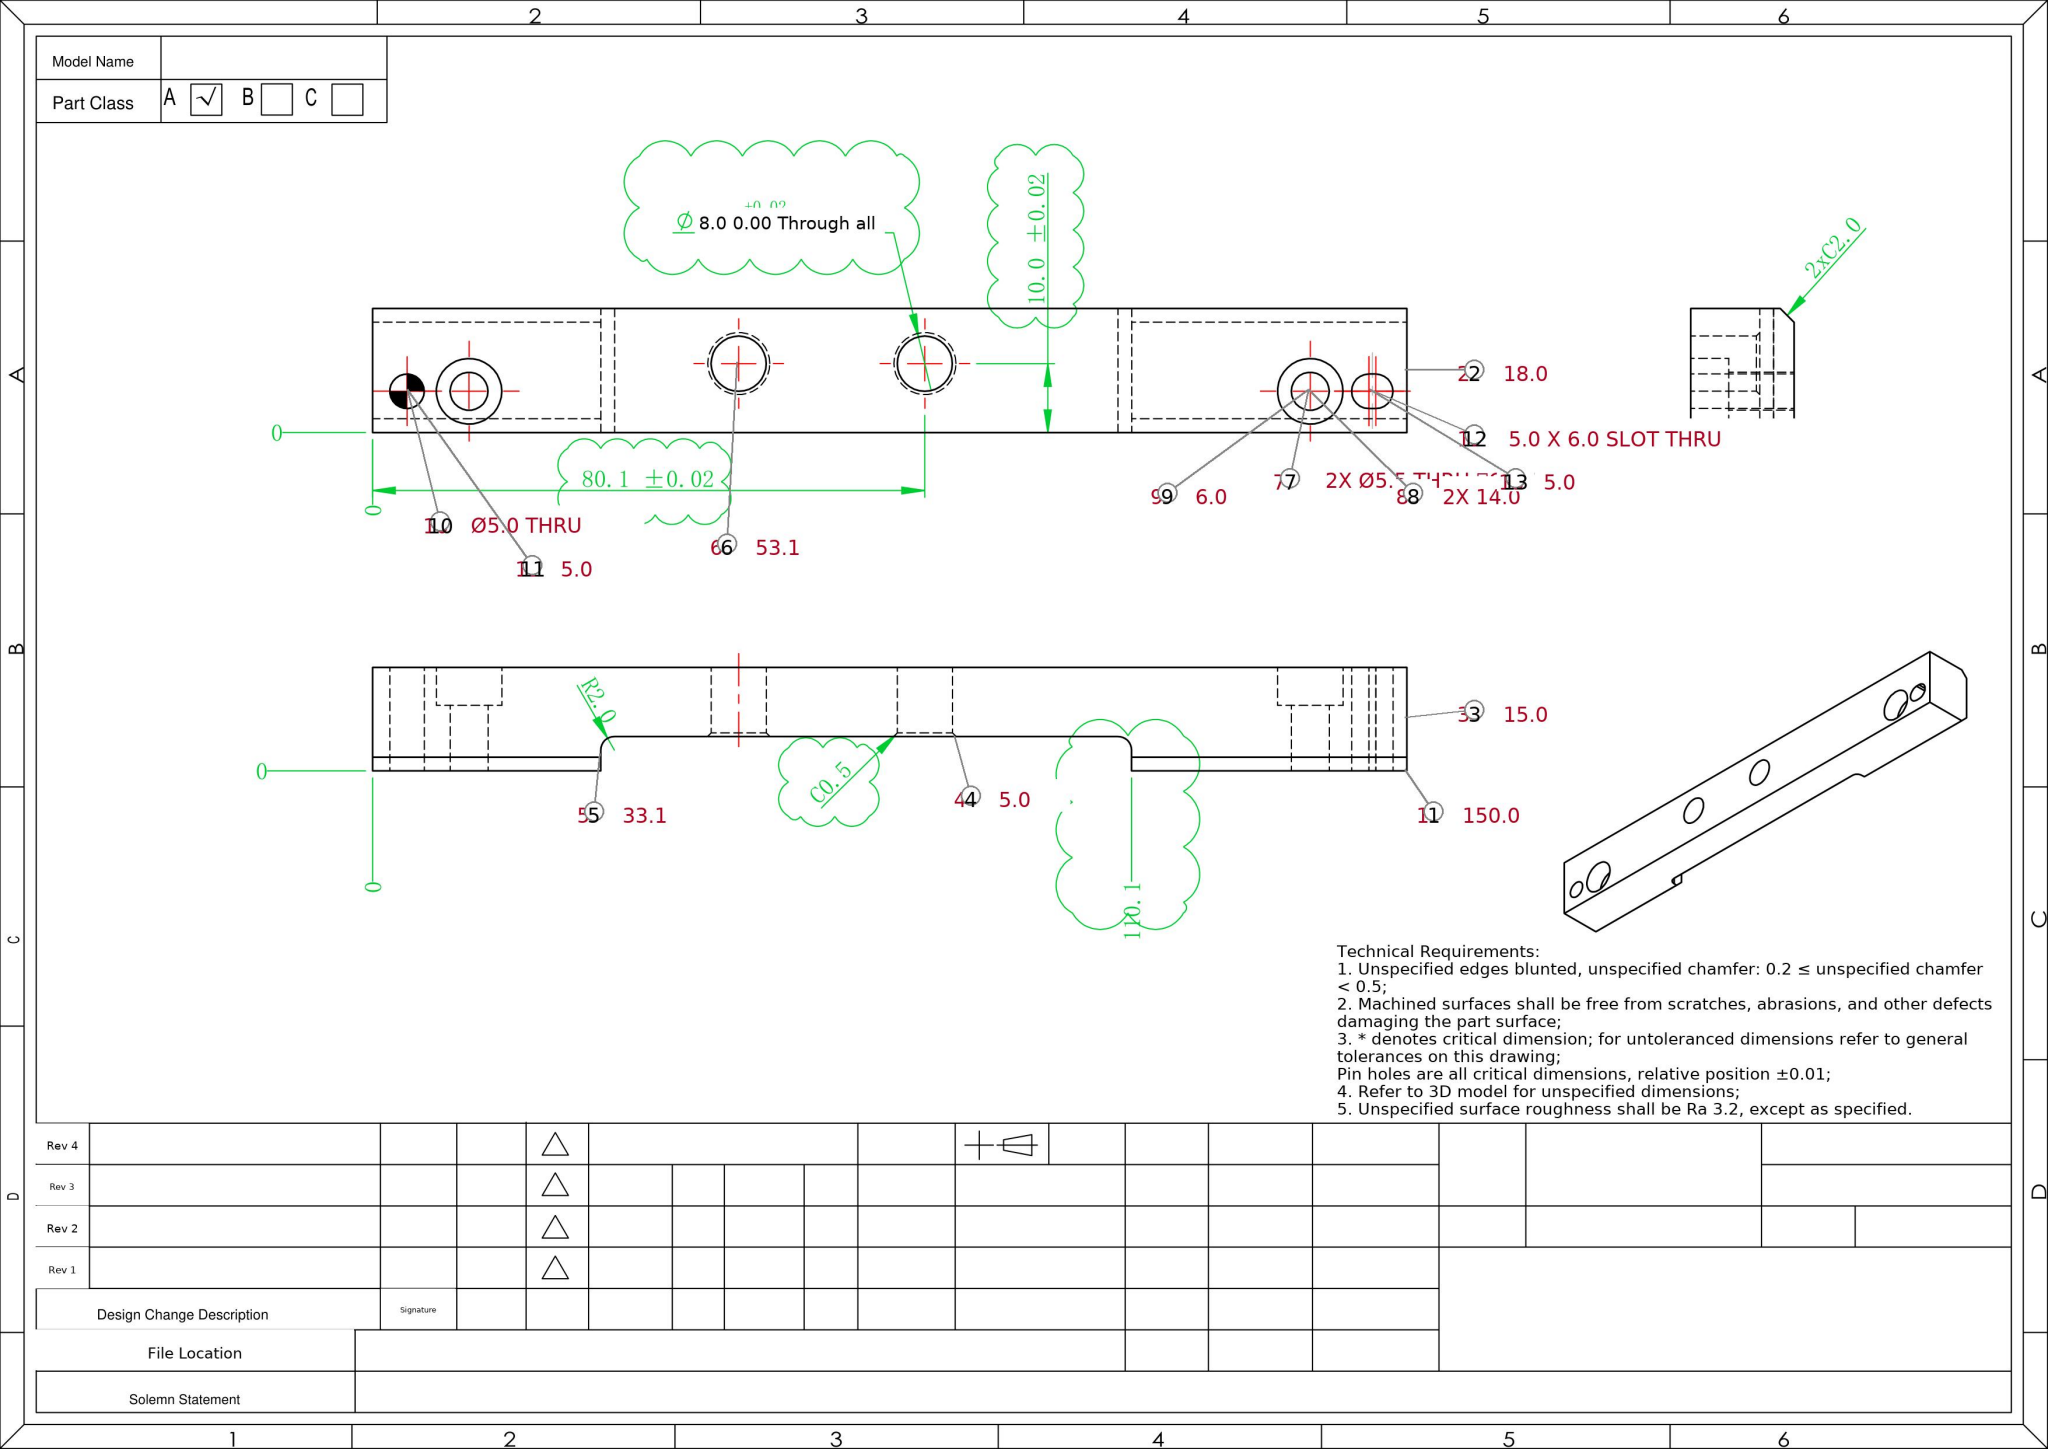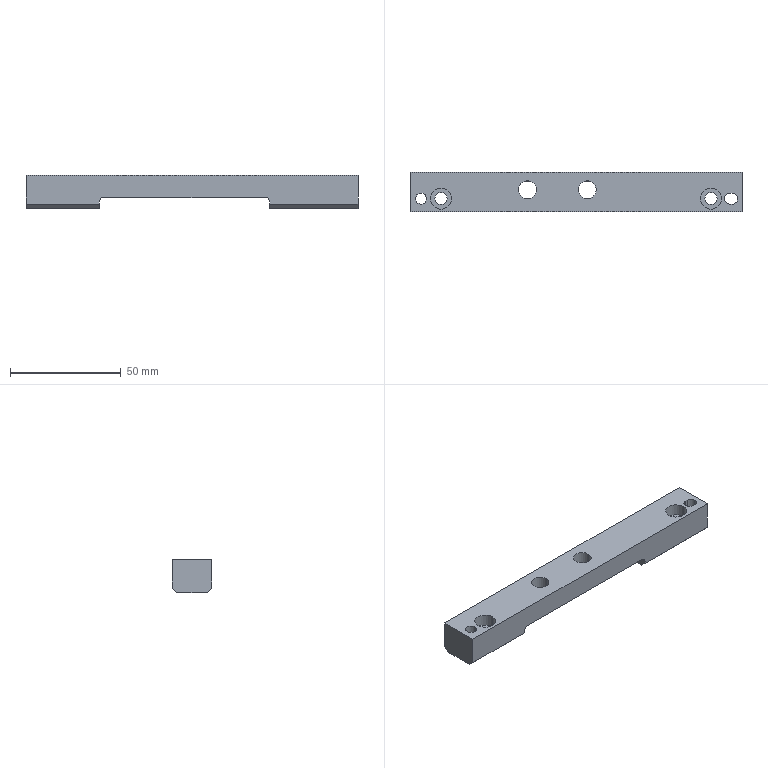Part | SolidWorks | mm | 1 solid | 41 faces | box 150 x 18 x 15 mm | volume 30402 mm3 | cylinder 19 | plane 18 | cone 4 | commonest cylinder face diameters 5 x5 8 x4 9.5 x4 5.5 x4 4 x2